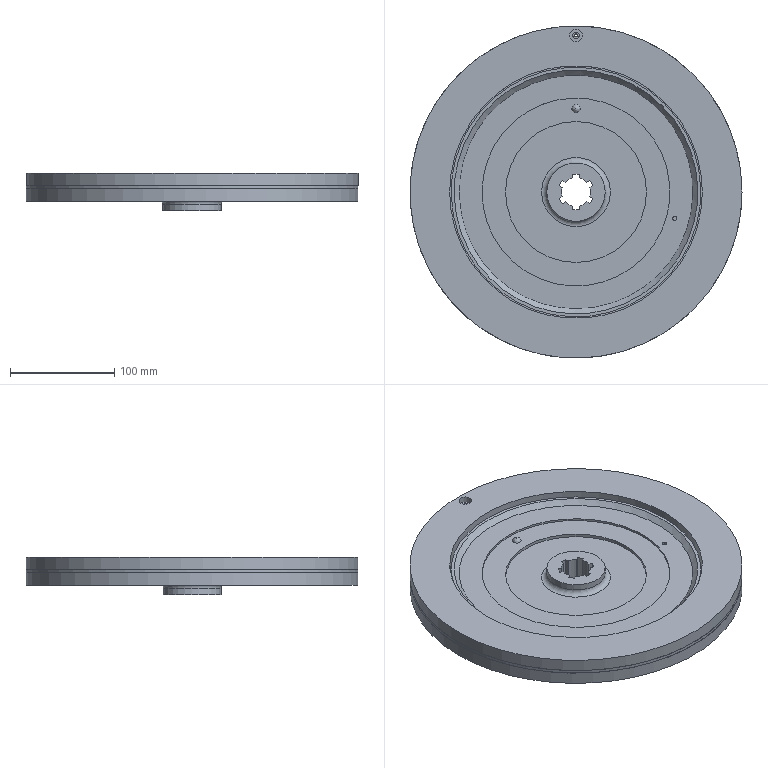Assembly | NX | mm | 7 component files | 7 solids | 79 faces | box 318 x 318 x 36 mm | volume 1320180 mm3 | plane 41 | cylinder 30 | cone 4 | spline 2 | torus 2 | commonest cylinder face diameters 28 x6 4 x3 318 x3 6 x3 5 x3 180 x2 242 x2 12 x2
Bill of materials:
unnamed part 1 | 1 |  | Flat circular disc with a cylindrical central hub sticking out from both faces. The hub has a through-bore with rectangular notches around it (spline-like or keyed). There is one small hole near the outer rim.
unnamed part 2 | 1 |  | Very thin flat annular plate (shim or washer-like) with a large central hole, a few small holes, and one narrow radial slit running in from the outer edge that ends in a small round hole.
unnamed part 3 | 2 |  | Thin flat ring with a chamfered or beveled outer edge, giving a trapezoidal cross-section in the side view. It has one small hole near the inner edge.
unnamed part 4 | 1 |  | Pin-like solid: a straight cylindrical shank with a dome-shaped (round) head of the same size at each end. It looks like a double round-head pin or a rivet in its set form.
unnamed part 5 | 2 |  | Flat ring with a rectangular cross-section and a large central opening, with one small through-hole near the outer edge.
Mates:
1. concentric | Rivet4x13L 1 edge | Support_plate_1 1 edge